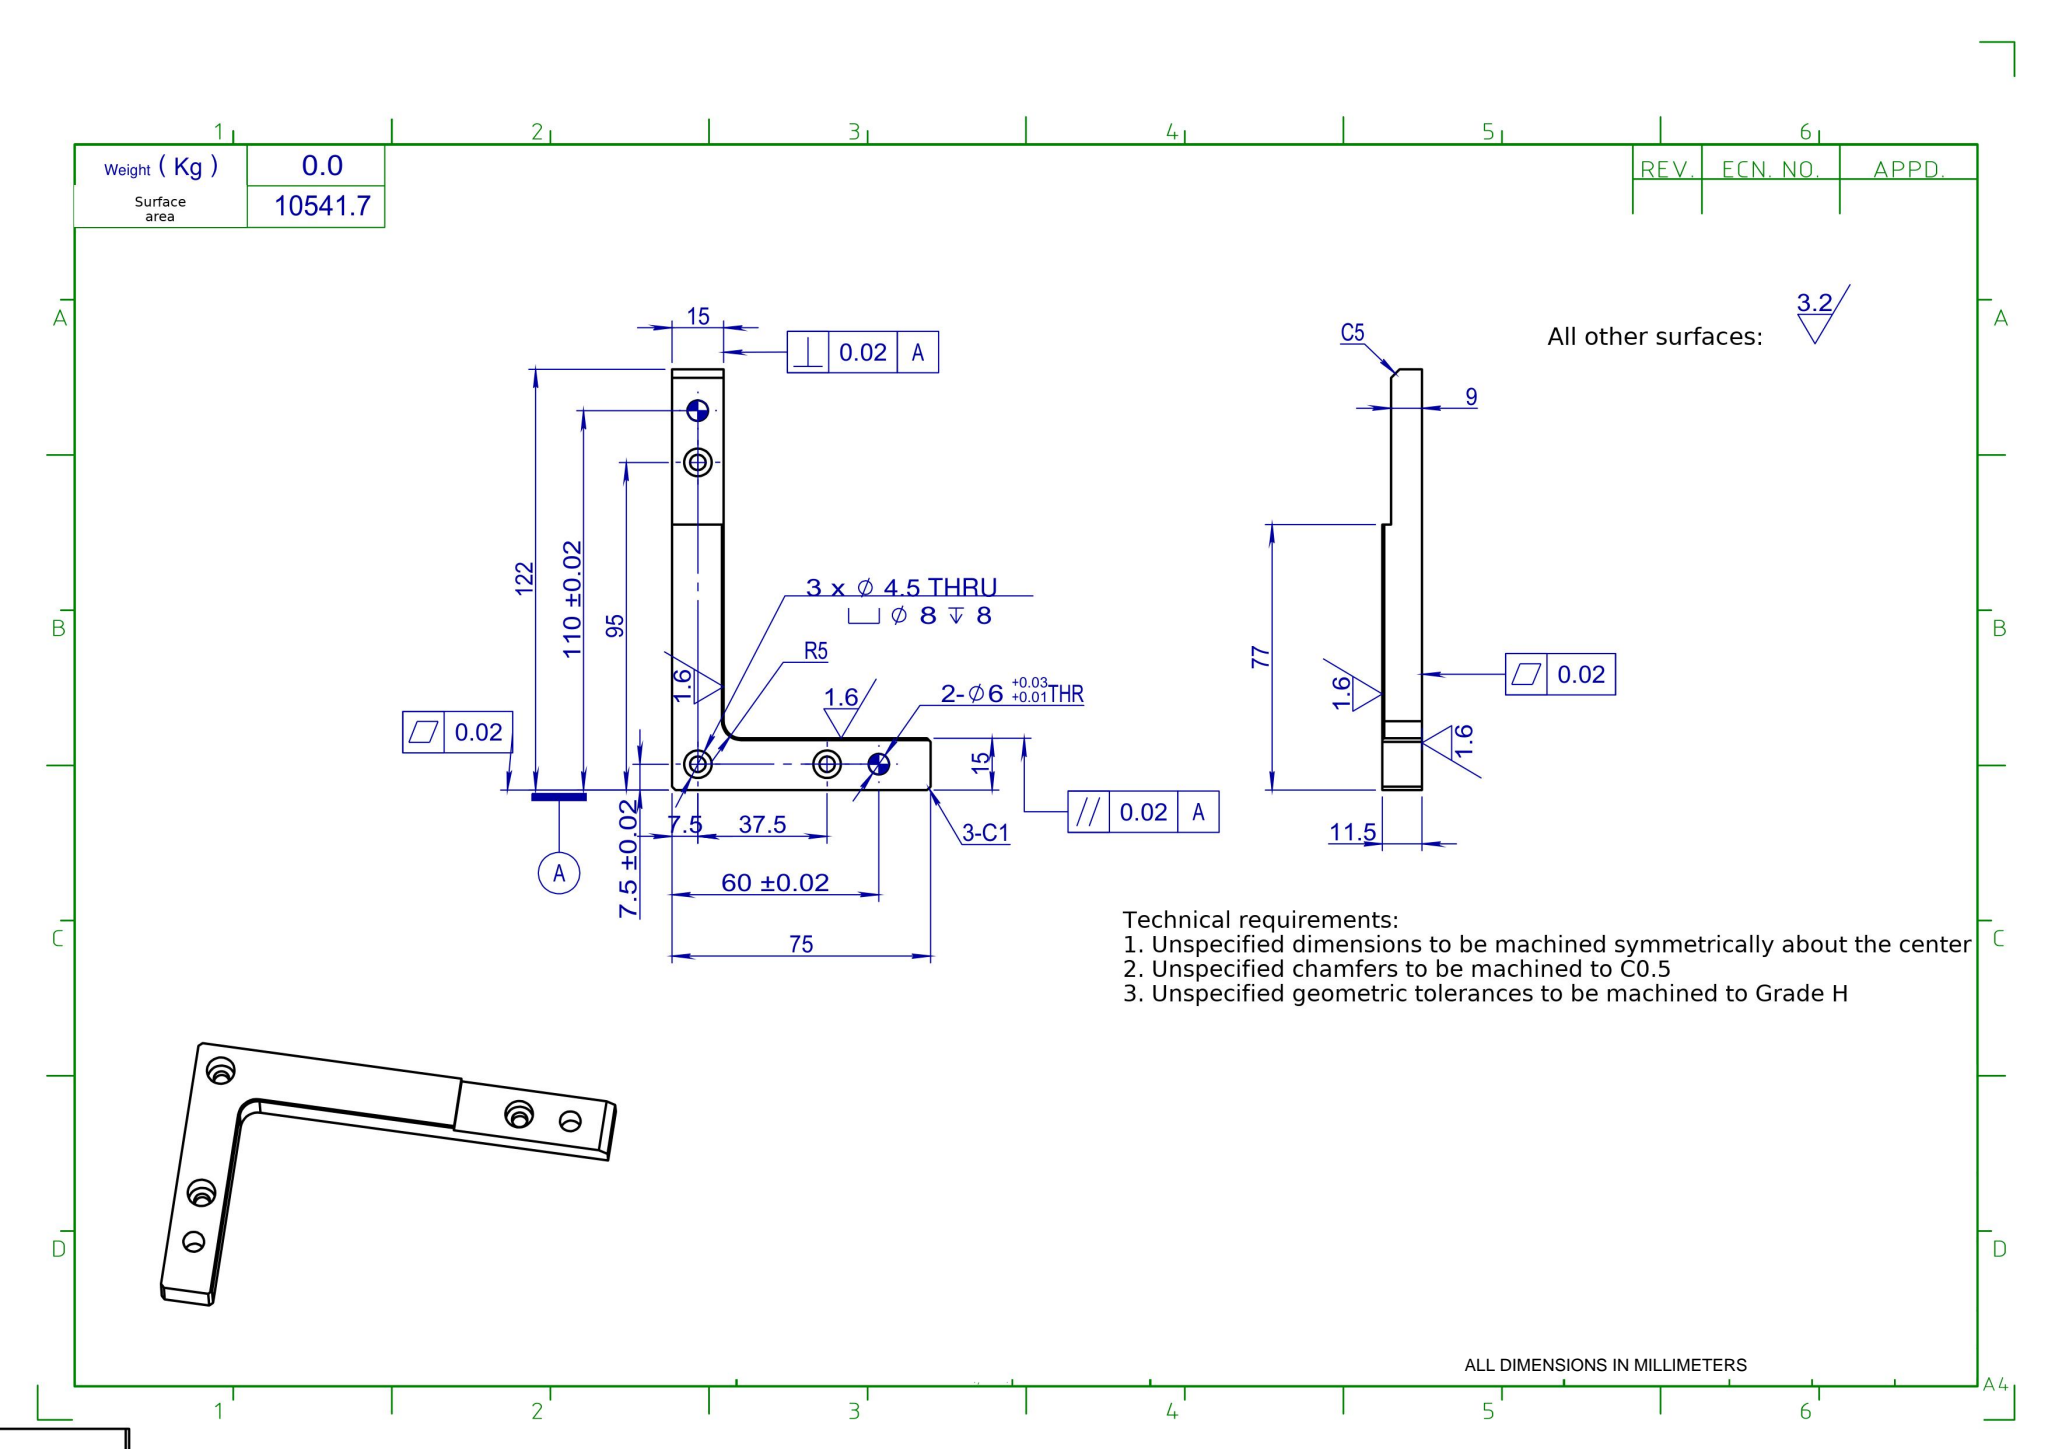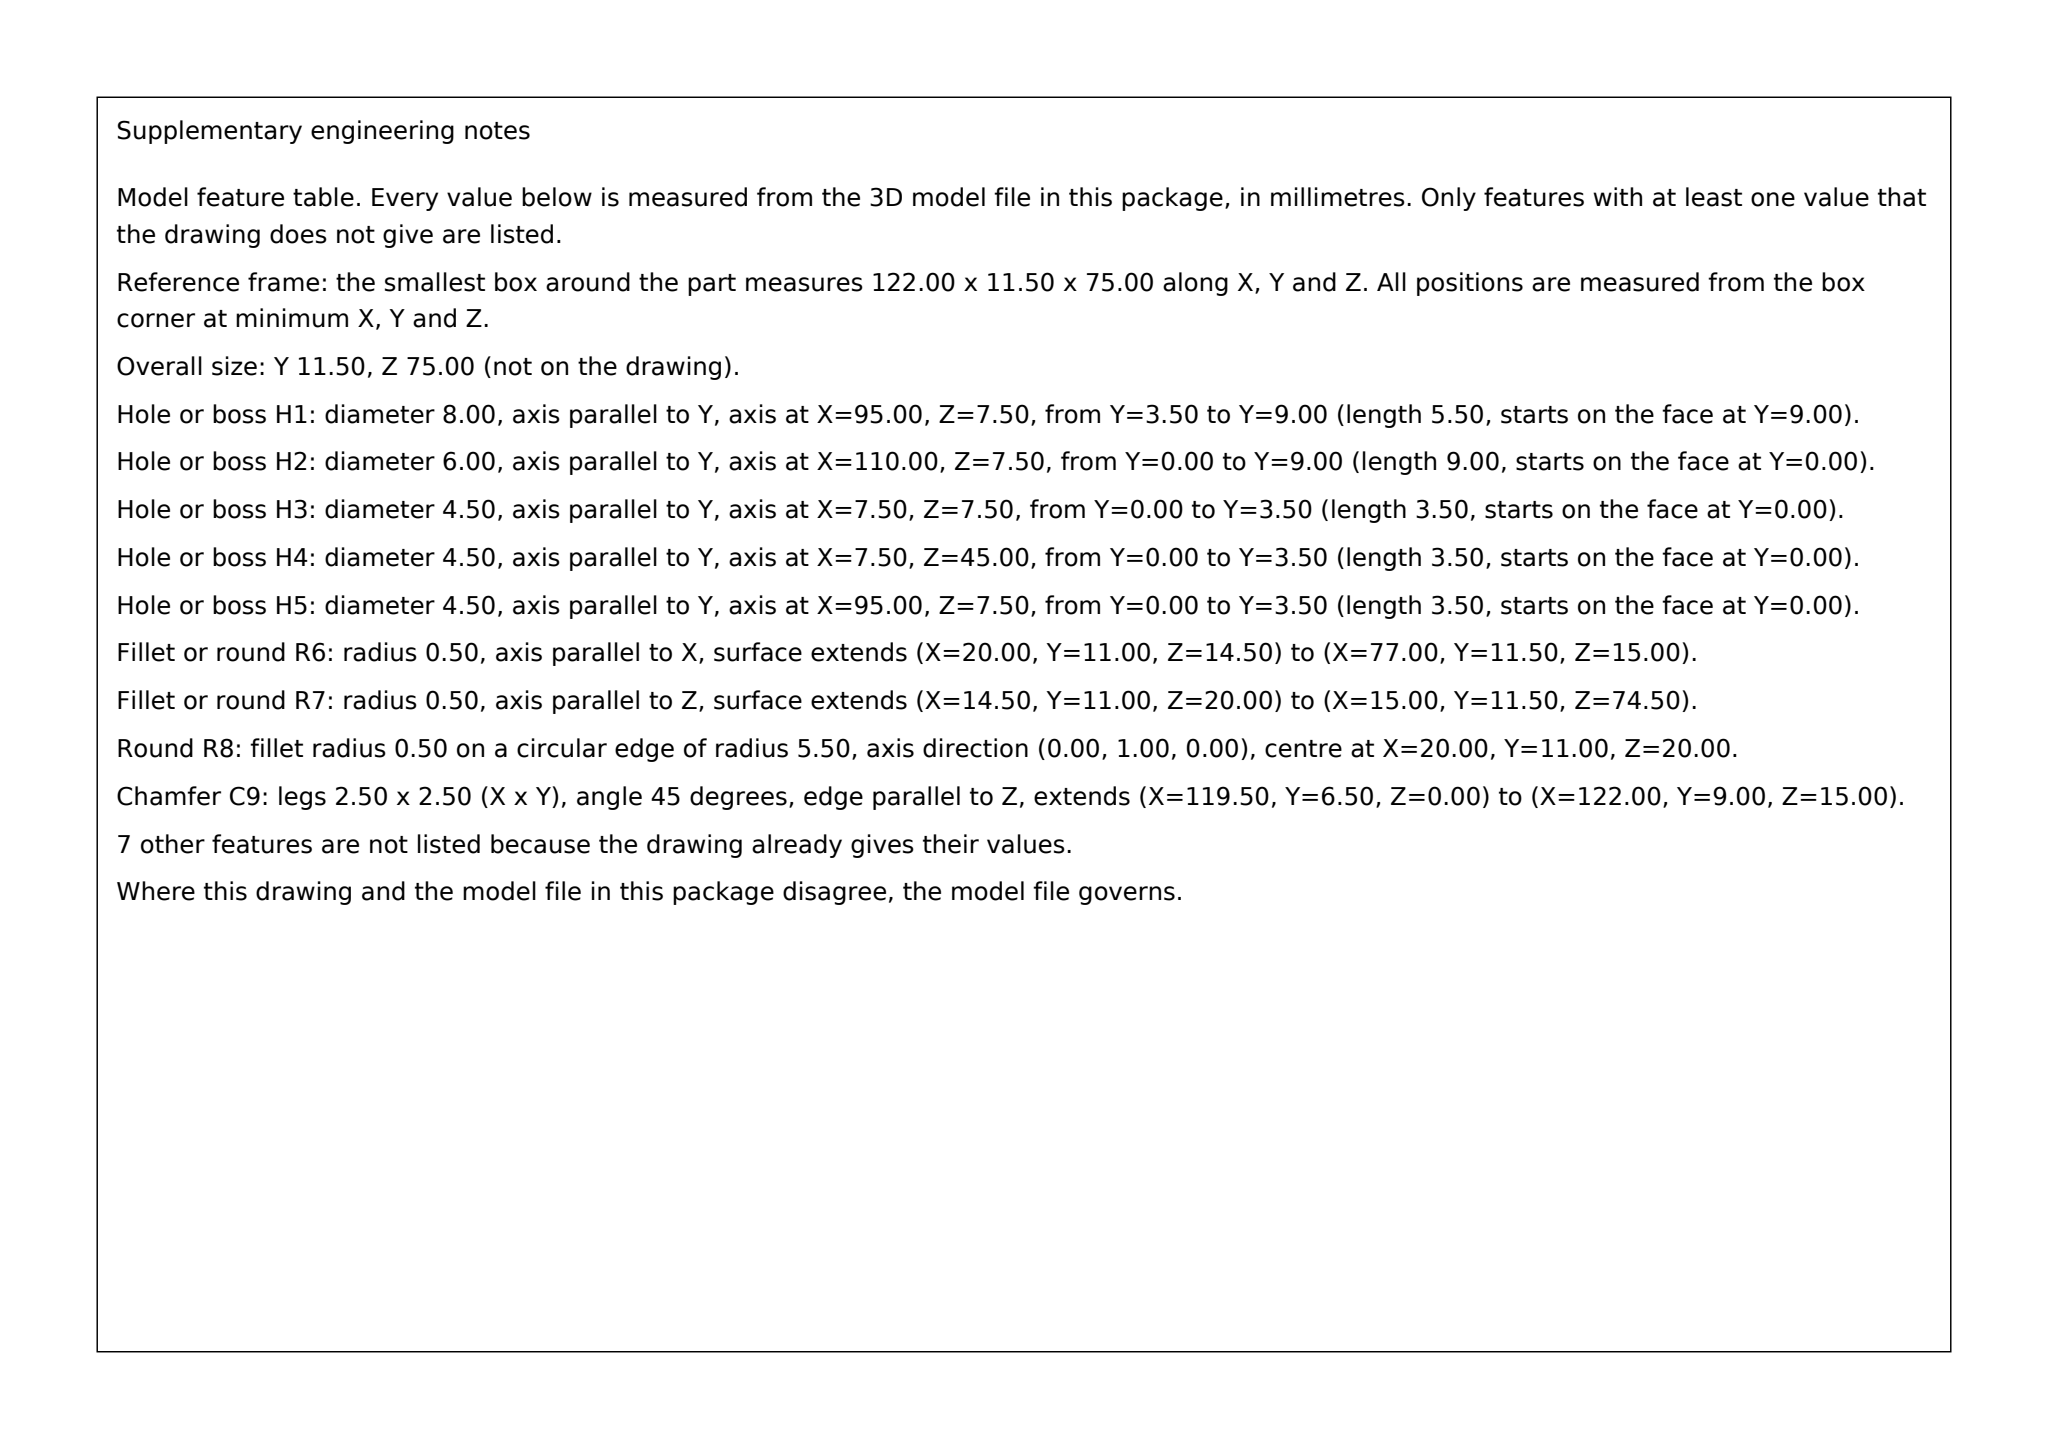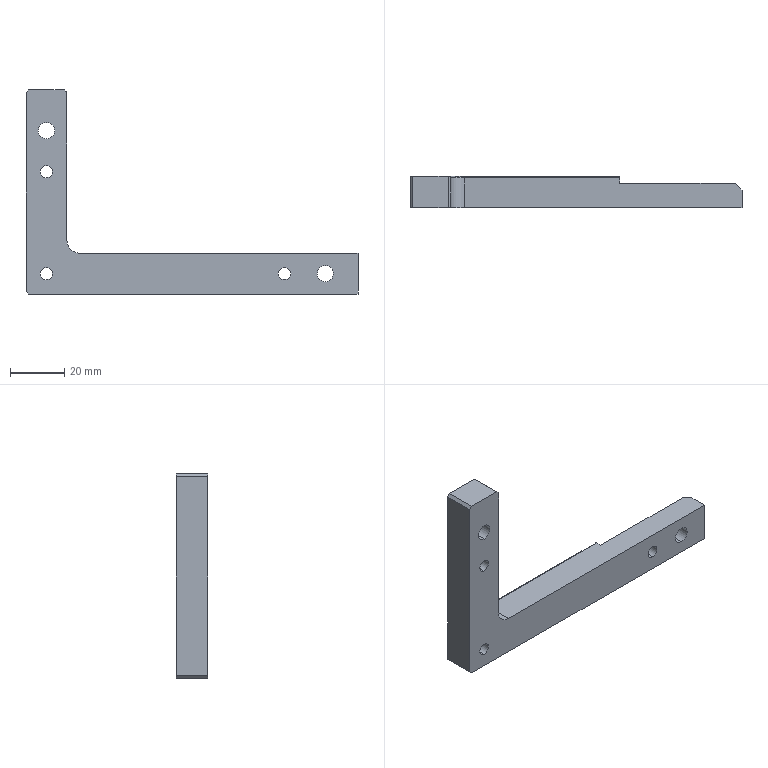Part | SolidWorks | mm | 1 solid | 37 faces | box 122 x 11.5 x 75 mm | volume 27871 mm3 | cylinder 19 | plane 17 | torus 1 | commonest cylinder face diameters 4.5 x6 8 x6 6 x4 1 x2 10 x1
build123d program:
from build123d import *

# Parameters (mm, degrees)
SKETCH1_W                                            = 140
SKETCH1_H                                            = 75
BOSS_EXTRUDE1_DEPTH                                  = 6
SKETCH2_W                                            = 125
SKETCH2_H                                            = 60
CUT_EXTRUDE1_DEPTH                                   = 80.638
BOSS_EXTRUDE2_DEPTH                                  = 5.5
FILLET1_R                                            = 5
CHAMFER1_SIZE                                        = 1
FILLET3_R                                            = 0.5
SKETCH7_R                                            = 3
CUT_EXTRUDE3_DEPTH                                   = 81.24
COUNTERBORE_FOR_M4_HEX_SOCKET_HEAD_CAP_S_D           = 4.5
COUNTERBORE_FOR_M4_HEX_SOCKET_HEAD_CAP_S_CBORE_D     = 8
COUNTERBORE_FOR_M4_HEX_SOCKET_HEAD_CAP_S_CBORE_DEPTH = 8
SKETCH10_W                                           = 18
SKETCH10_H                                           = 15
CUT_EXTRUDE4_DEPTH                                   = 81.24
CUT_EXTRUDE5_DEPTH                                   = 103.767
SKETCH12_W                                           = 45
SKETCH12_H                                           = 15
CUT_EXTRUDE6_DEPTH                                   = 2.5


with BuildPart() as part:
    # Sketch1 → Boss-Extrude1 (new body)
    with BuildSketch(Plane(origin=(0, 0, 0), x_dir=(1, 0, 0), z_dir=(0, 1, 0))):
        Rectangle(SKETCH1_W, SKETCH1_H)
    extrude(amount=BOSS_EXTRUDE1_DEPTH)

    # Sketch2 → Cut-Extrude1 (cut, through all)
    with BuildSketch(Plane(origin=(0, 6, 0), x_dir=(1, 0, 0), z_dir=(0, 1, 0))):
        with Locations((7.5, -7.5)):
            Rectangle(SKETCH2_W, SKETCH2_H)
    extrude(amount=-CUT_EXTRUDE1_DEPTH, mode=Mode.SUBTRACT)

    # Sketch3 → Boss-Extrude2 (add)
    with BuildSketch(Plane.XZ):
        Polygon((70, -22.5), (-55, -22.5), (-55, 37.5), (-70, 37.5), (-70, -37.5), (70, -37.5), align=None)
    extrude(amount=BOSS_EXTRUDE2_DEPTH)

    # Fillet1
    fillet1_edges = [part.edges().sort_by_distance(p)[0] for p in [
        (-55, 0.25, -22.5),
    ]]
    fillet(fillet1_edges, radius=FILLET1_R)

    # Chamfer1
    chamfer1_edges = [part.edges().sort_by_distance(p)[0] for p in [
        (70, 0.25, -22.5),
        (-55, 0.25, 37.5),
        (-70, 0.25, -37.5),
        (70, 0.25, -37.5),
        (-70, 0.25, 37.5),
    ]]
    chamfer(chamfer1_edges, length=CHAMFER1_SIZE)

    # Fillet3
    fillet3_edges = [part.edges().sort_by_distance(p)[0] for p in [
        (-55, 6, 9.5),
        (-53.536, 6, -21.036),
        (9.5, 6, -22.5),
    ]]
    fillet(fillet3_edges, radius=FILLET3_R)

    # Sketch7 → Cut-Extrude3 (cut, through all)
    with BuildSketch(Plane(origin=(0, 6, 0), x_dir=(1, 0, 0), z_dir=(0, 1, 0))):
        with Locations(Location((40, 30, 0), (0, 0, 270))):
            Circle(SKETCH7_R)
        with Locations(Location((-62.5, -22.5, 0), (0, 0, 270))):
            Circle(SKETCH7_R)
    extrude(amount=-CUT_EXTRUDE3_DEPTH, mode=Mode.SUBTRACT)

    # Counterbore for M4 Hex Socket Head Cap S (through all)
    with Locations(Plane(origin=(0, 6, 0), x_dir=(1, 0, 0), z_dir=(0, 1, 0))):
        with Locations((25, 30), (-62.5, -7.5), (-62.5, 30)):
            CounterBoreHole(COUNTERBORE_FOR_M4_HEX_SOCKET_HEAD_CAP_S_D / 2, COUNTERBORE_FOR_M4_HEX_SOCKET_HEAD_CAP_S_CBORE_D / 2, COUNTERBORE_FOR_M4_HEX_SOCKET_HEAD_CAP_S_CBORE_DEPTH)

    # Sketch10 → Cut-Extrude4 (cut, through all)
    with BuildSketch(Plane(origin=(0, 6, 0), x_dir=(1, 0, 0), z_dir=(0, 1, 0))):
        with Locations((61, 30)):
            Rectangle(SKETCH10_W, SKETCH10_H)
    extrude(amount=-CUT_EXTRUDE4_DEPTH, mode=Mode.SUBTRACT)

    # Sketch11 → Cut-Extrude5 (cut, through all)
    with BuildSketch(Plane(origin=(0, 0, -37.5), x_dir=(-1, 0, 0), z_dir=(0, 0, -1))):
        Polygon((-47, 6), (-52, 1), (-52, 6), align=None)
    extrude(amount=-CUT_EXTRUDE5_DEPTH, mode=Mode.SUBTRACT)

    # Sketch12 → Cut-Extrude6 (cut)
    with BuildSketch(Plane(origin=(0, 6, 0), x_dir=(1, 0, 0), z_dir=(0, 1, 0))):
        with Locations((29.5, 30)):
            Rectangle(SKETCH12_W, SKETCH12_H)
    extrude(amount=-CUT_EXTRUDE6_DEPTH, mode=Mode.SUBTRACT)


solid = part.part